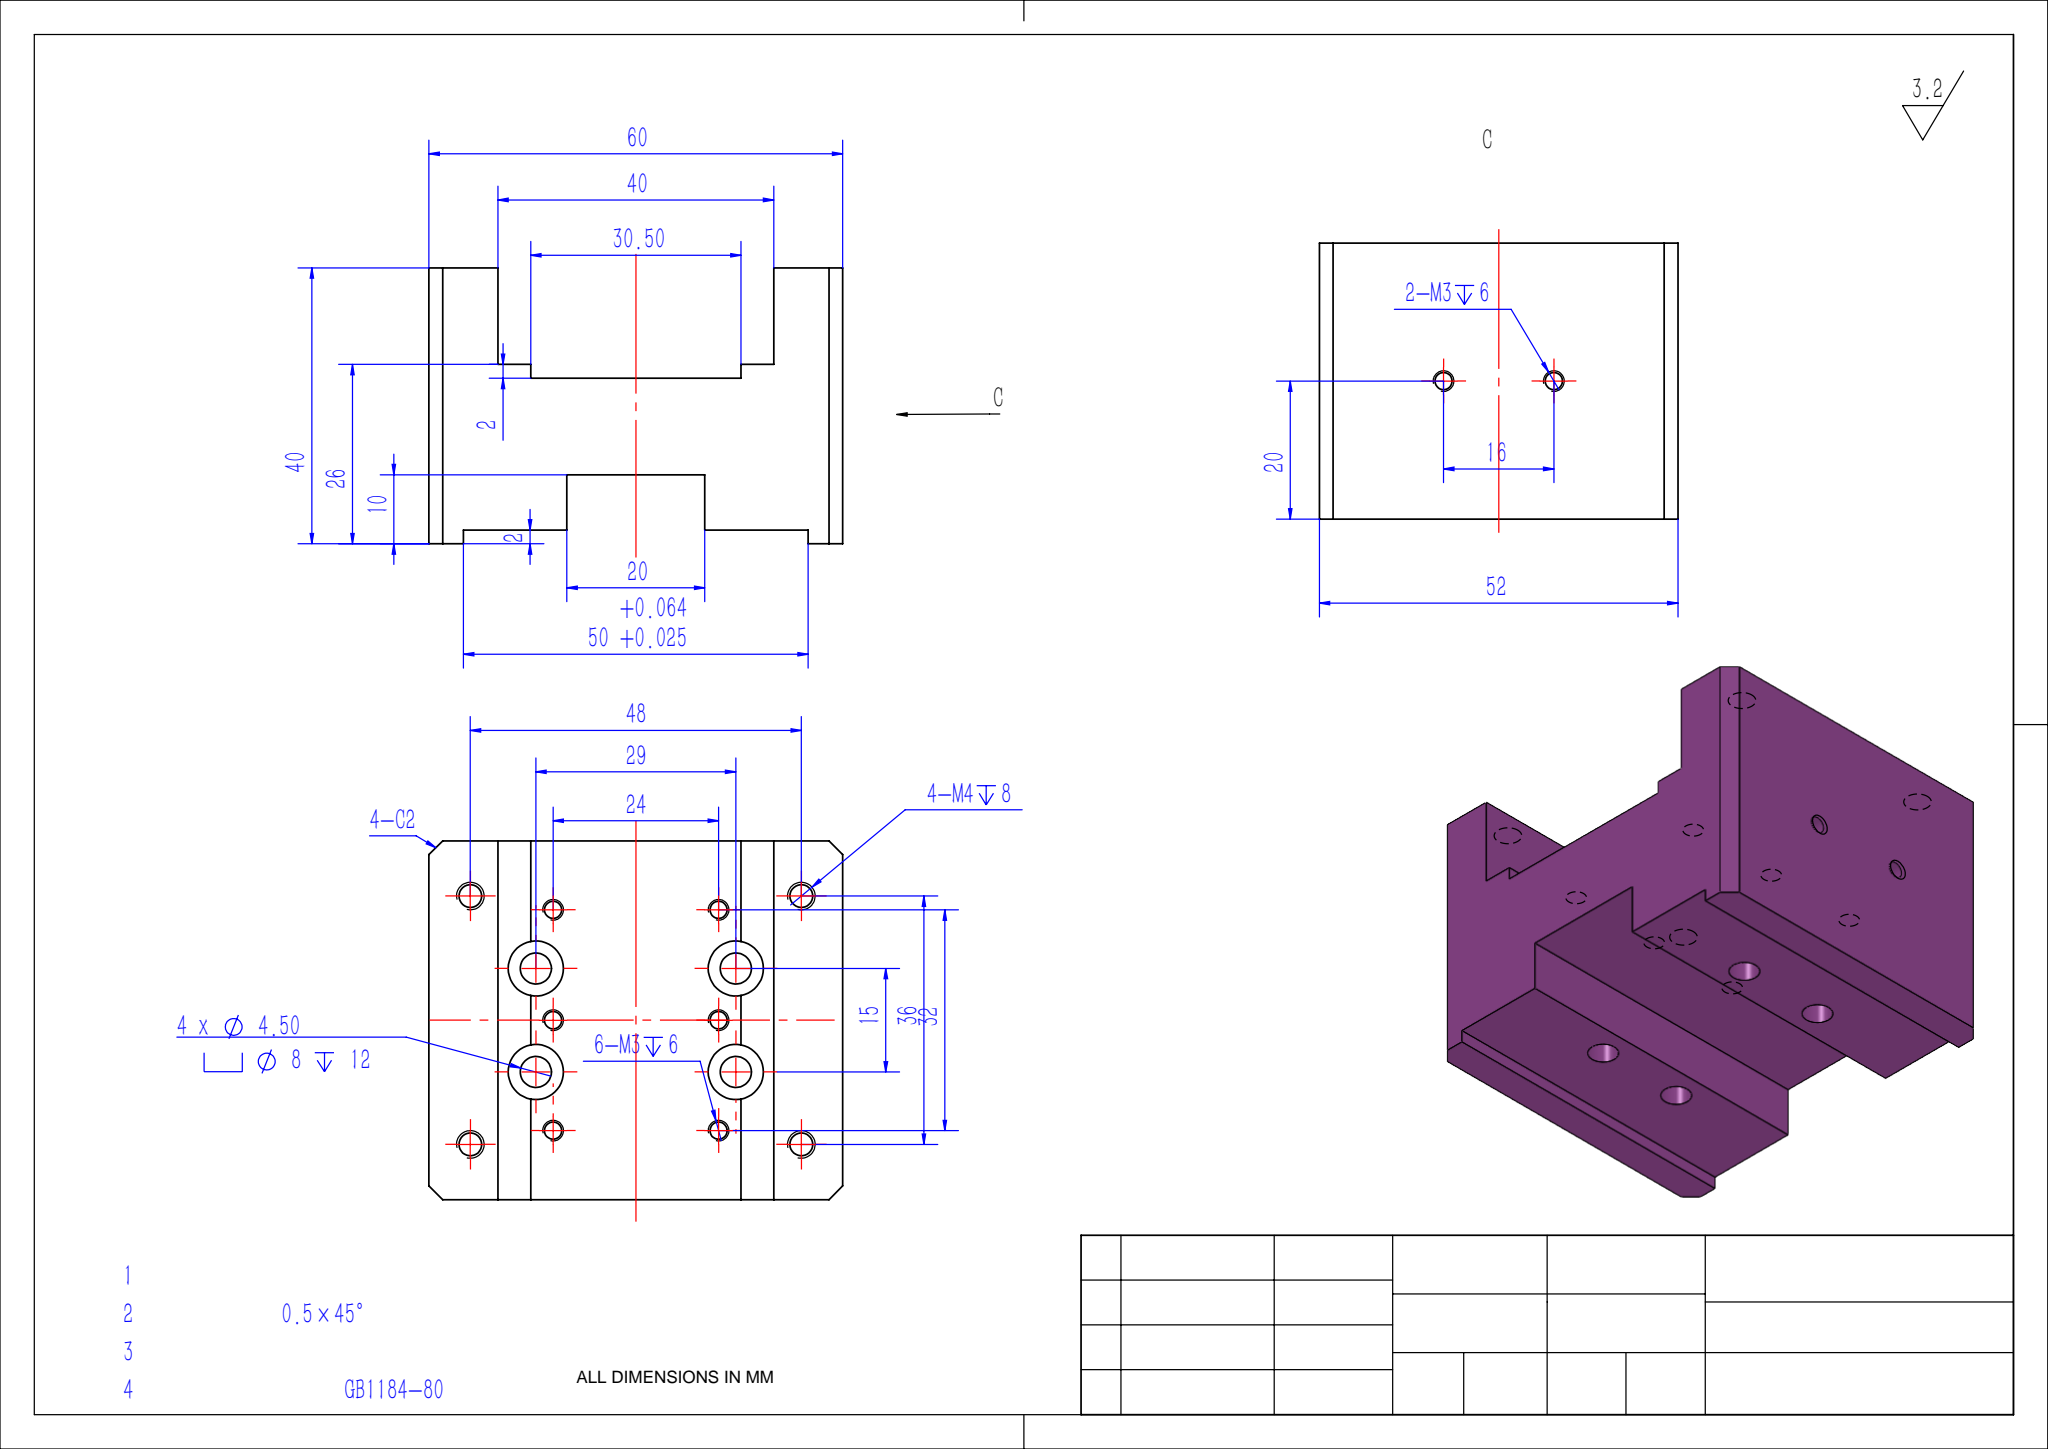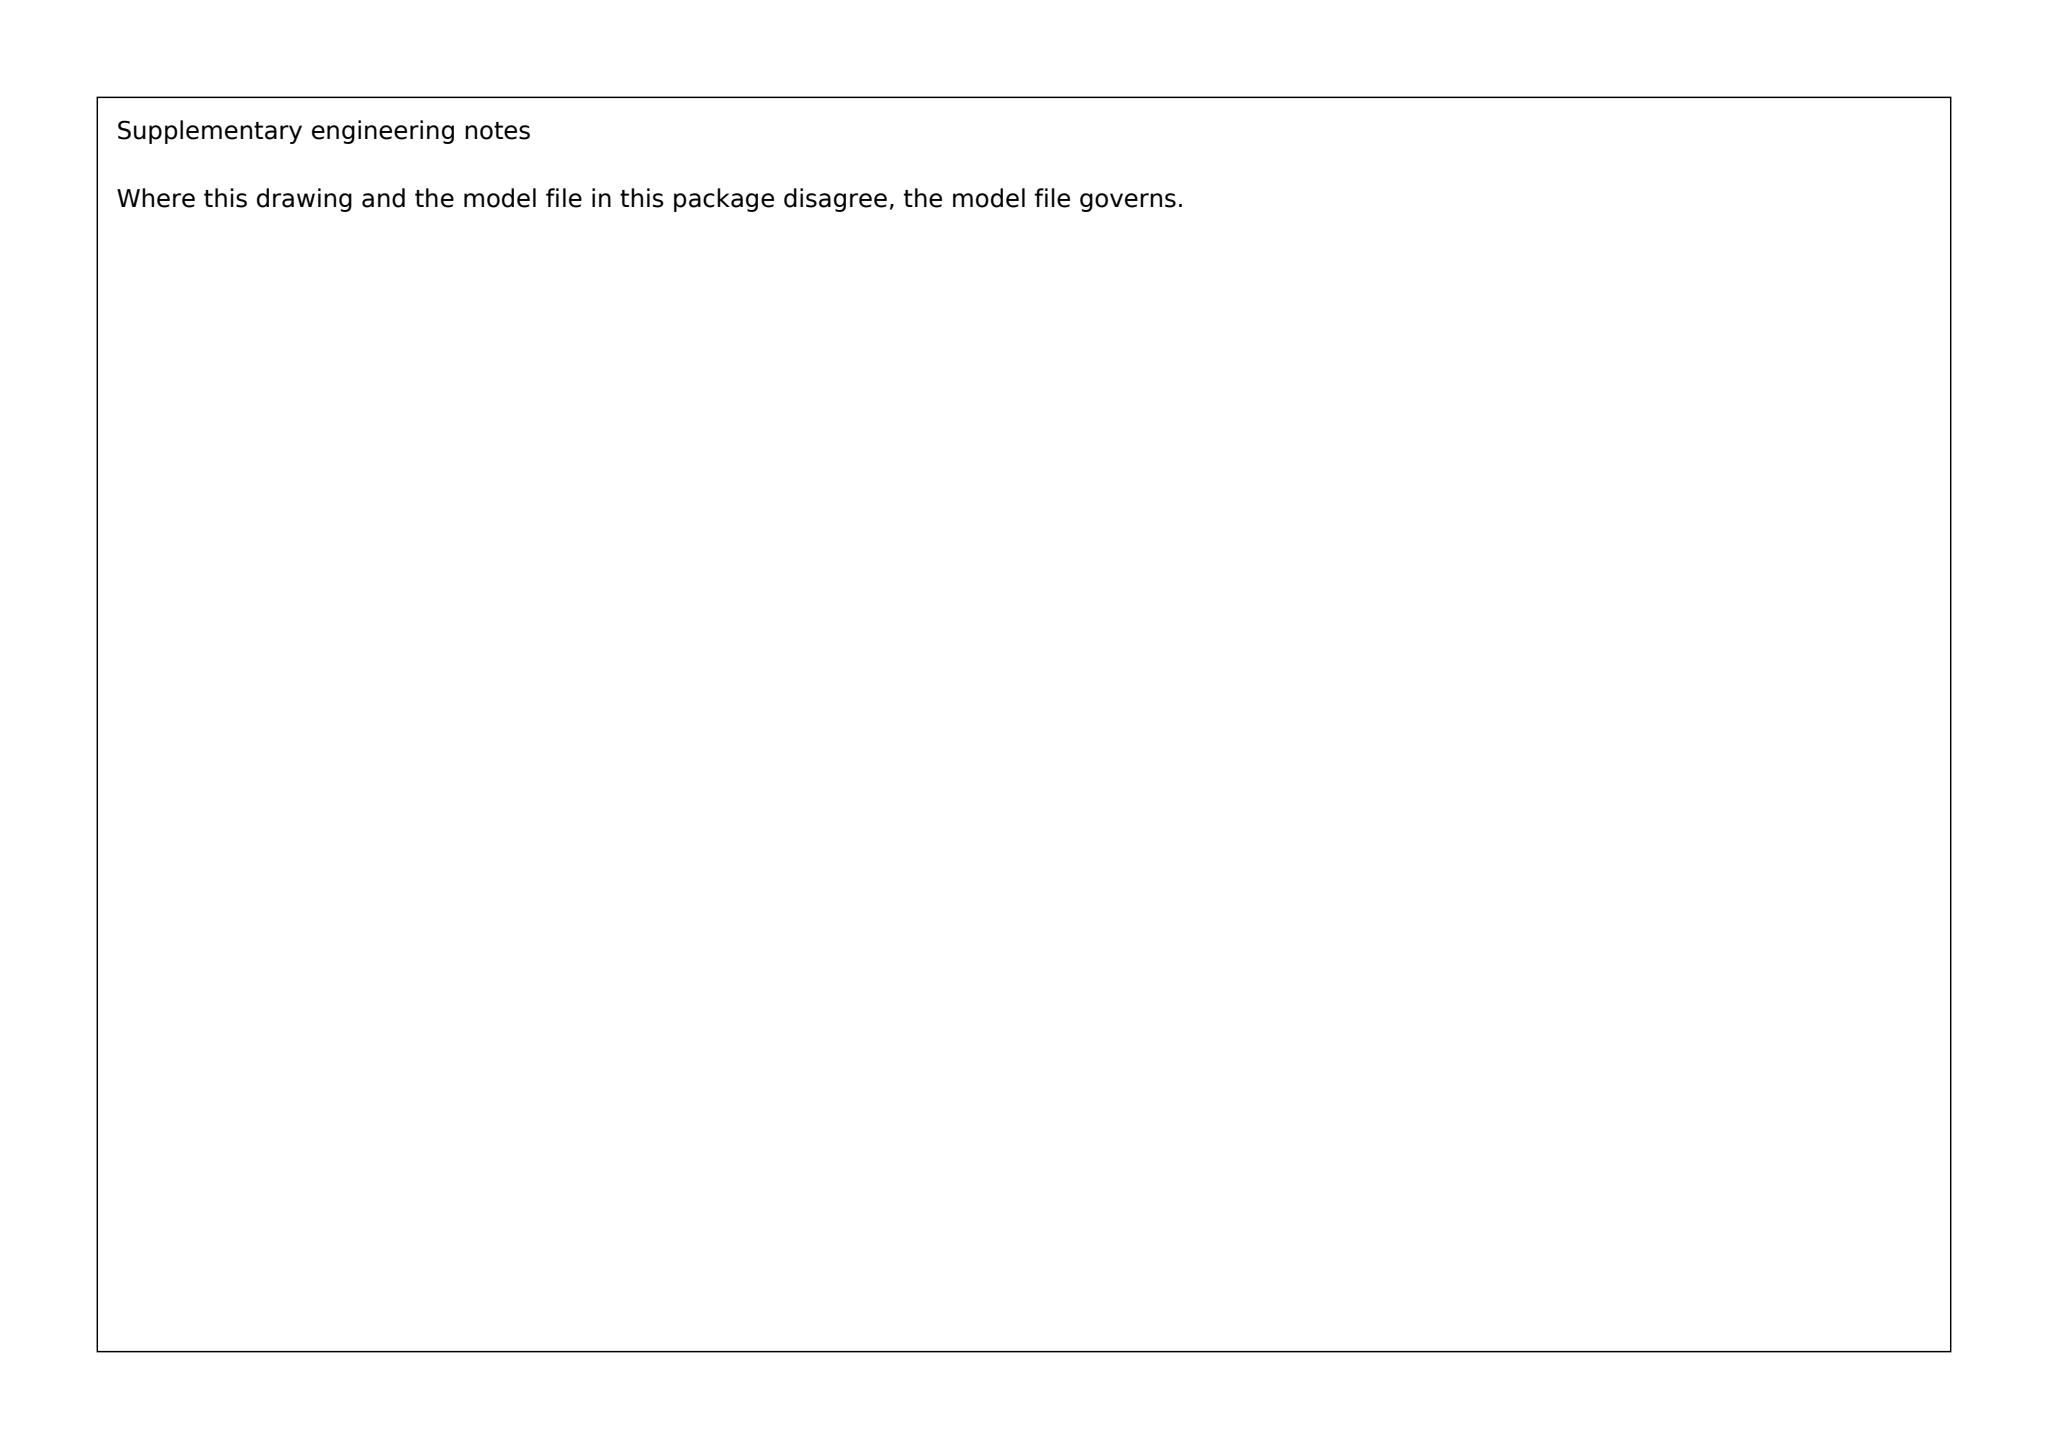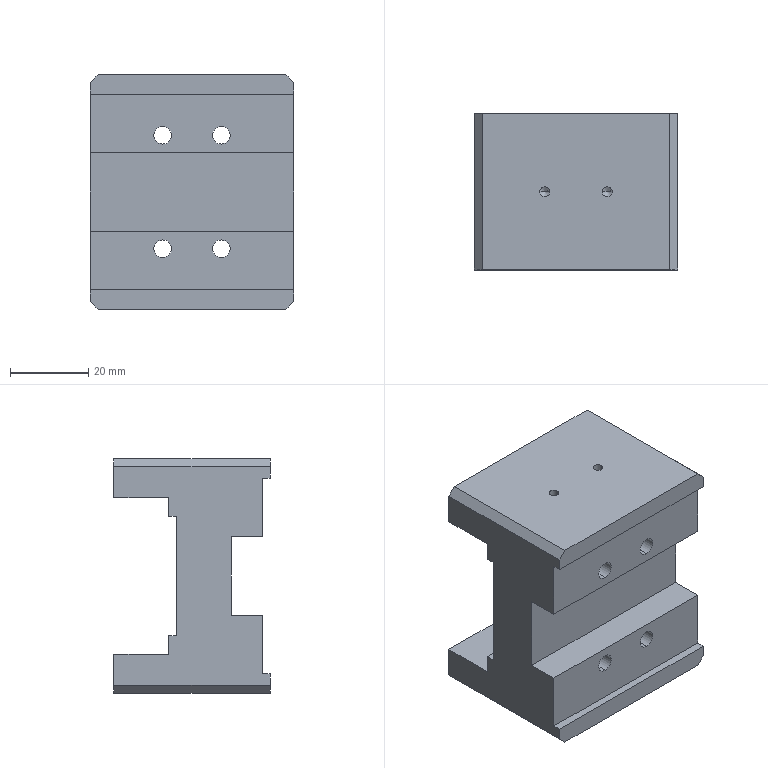Part | SolidWorks | mm | 1 solid | 98 faces | box 52 x 40 x 60 mm | volume 75079 mm3 | cylinder 40 | plane 34 | cone 24 | commonest cylinder face diameters 2.5 x16 3.3 x8 4.5 x8 8 x8
build123d program:
from build123d import *

# Parameters (mm, degrees)
SKETCH1_W                                         = 52
SKETCH1_H                                         = 60
BOSS_EXTRUDE1_DEPTH                               = 40
SKETCH2_W                                         = 52
SKETCH2_H                                         = 50
CUT_EXTRUDE1_DEPTH                                = 2
SKETCH3_W                                         = 52
SKETCH3_H                                         = 20
CUT_EXTRUDE2_DEPTH                                = 8
HOLE_SIZE_ACCORDING_TO_HEXAGON_SOCKET_D           = 4.5
HOLE_SIZE_ACCORDING_TO_HEXAGON_SOCKET_CBORE_D     = 8
HOLE_SIZE_ACCORDING_TO_HEXAGON_SOCKET_CBORE_DEPTH = 26
SKETCH7_W                                         = 52
SKETCH7_H                                         = 40
CUT_EXTRUDE3_DEPTH                                = 14
SKETCH9_W                                         = 52
SKETCH9_H                                         = 30.5
CUT_EXTRUDE4_DEPTH                                = 2
M3_TAPPED_HOLE1_D                                 = 2.5
M3_TAPPED_HOLE1_DEPTH                             = 7.5
M3_TAPPED_HOLE1_TIP                               = 0.7511
CHAMFER1_SIZE                                     = 2
M4_TAPPED_HOLE1_D                                 = 3.3
M4_TAPPED_HOLE1_DEPTH                             = 10.1
M4_TAPPED_HOLE1_TIP                               = 0.9914
M3_TAPPED_HOLE2_D                                 = 2.5
M3_TAPPED_HOLE2_DEPTH                             = 7.5
M3_TAPPED_HOLE2_TIP                               = 0.7511


with BuildPart() as part:
    # Sketch1 → Boss-Extrude1 (new body)
    with BuildSketch(Plane(origin=(0, 0, 0), x_dir=(1, 0, 0), z_dir=(0, 1, 0))):
        Rectangle(SKETCH1_W, SKETCH1_H)
    extrude(amount=BOSS_EXTRUDE1_DEPTH)

    # Sketch2 → Cut-Extrude1 (cut)
    with BuildSketch(Plane.XZ):
        Rectangle(SKETCH2_W, SKETCH2_H)
    extrude(amount=-CUT_EXTRUDE1_DEPTH, mode=Mode.SUBTRACT)

    # Sketch3 → Cut-Extrude2 (cut)
    with BuildSketch(Plane.XZ.offset(-2)):
        Rectangle(SKETCH3_W, SKETCH3_H)
    extrude(amount=-CUT_EXTRUDE2_DEPTH, mode=Mode.SUBTRACT)

    # Hole Size _ according to_ Hexagon Socket (through all)
    with Locations(Plane(origin=(0, 40, 0), x_dir=(1, 0, 0), z_dir=(0, 1, 0))):
        with Locations((-7.5, 14.5), (7.5, 14.5), (-7.5, -14.5), (7.5, -14.5)):
            CounterBoreHole(HOLE_SIZE_ACCORDING_TO_HEXAGON_SOCKET_D / 2, HOLE_SIZE_ACCORDING_TO_HEXAGON_SOCKET_CBORE_D / 2, HOLE_SIZE_ACCORDING_TO_HEXAGON_SOCKET_CBORE_DEPTH)

    # Sketch7 → Cut-Extrude3 (cut)
    with BuildSketch(Plane(origin=(0, 40, 0), x_dir=(1, 0, 0), z_dir=(0, 1, 0))):
        Rectangle(SKETCH7_W, SKETCH7_H)
    extrude(amount=-CUT_EXTRUDE3_DEPTH, mode=Mode.SUBTRACT)

    # Sketch9 → Cut-Extrude4 (cut)
    with BuildSketch(Plane(origin=(0, 26, 0), x_dir=(1, 0, 0), z_dir=(0, 1, 0))):
        Rectangle(SKETCH9_W, SKETCH9_H)
    extrude(amount=-CUT_EXTRUDE4_DEPTH, mode=Mode.SUBTRACT)

    # M3 Tapped Hole1
    with Locations(Plane(origin=(0, 24, 0), x_dir=(1, 0, 0), z_dir=(0, 1, 0))):
        with Locations((-16, 12), (-16, -12), (0, -12), (0, 12), (16, 12), (16, -12)):
            Hole(M3_TAPPED_HOLE1_D / 2, depth=M3_TAPPED_HOLE1_DEPTH)
            with Locations((0, 0, -(M3_TAPPED_HOLE1_DEPTH + M3_TAPPED_HOLE1_TIP / 2))):  # 118° drill point
                Cone(0, M3_TAPPED_HOLE1_D / 2, M3_TAPPED_HOLE1_TIP, mode=Mode.SUBTRACT)

    # Chamfer1
    chamfer1_edges = [part.edges().sort_by_distance(p)[0] for p in [
        (-26, 20, -30),
        (26, 20, -30),
        (26, 20, 30),
        (-26, 20, 30),
    ]]
    chamfer(chamfer1_edges, length=CHAMFER1_SIZE)

    # M4 Tapped Hole1
    with Locations(Plane(origin=(0, 40, 0), x_dir=(1, 0, 0), z_dir=(0, 1, 0))):
        with Locations((-18, -24), (18, -24), (18, 24), (-18, 24)):
            Hole(M4_TAPPED_HOLE1_D / 2, depth=M4_TAPPED_HOLE1_DEPTH)
            with Locations((0, 0, -(M4_TAPPED_HOLE1_DEPTH + M4_TAPPED_HOLE1_TIP / 2))):  # 118° drill point
                Cone(0, M4_TAPPED_HOLE1_D / 2, M4_TAPPED_HOLE1_TIP, mode=Mode.SUBTRACT)

    # M3 Tapped Hole2
    with Locations(Plane.XY.offset(30)):
        with Locations((-8, 20), (8, 20)):
            Hole(M3_TAPPED_HOLE2_D / 2, depth=M3_TAPPED_HOLE2_DEPTH)
            with Locations((0, 0, -(M3_TAPPED_HOLE2_DEPTH + M3_TAPPED_HOLE2_TIP / 2))):  # 118° drill point
                Cone(0, M3_TAPPED_HOLE2_D / 2, M3_TAPPED_HOLE2_TIP, mode=Mode.SUBTRACT)


solid = part.part